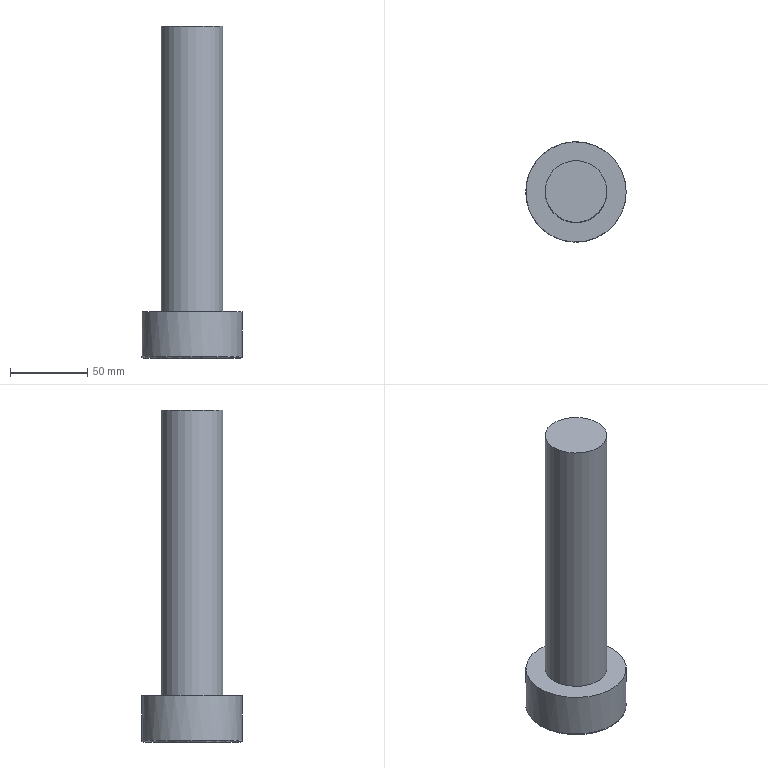Component | NX | TRANSITION_ACTUATOR_FLANGE_SCREW | 1 solid | 31 faces | volume 316501 mm3 | plane 16 | cylinder 14 | torus 1 | commonest cylinder face diameters 2 x12 65 x1 40 x1